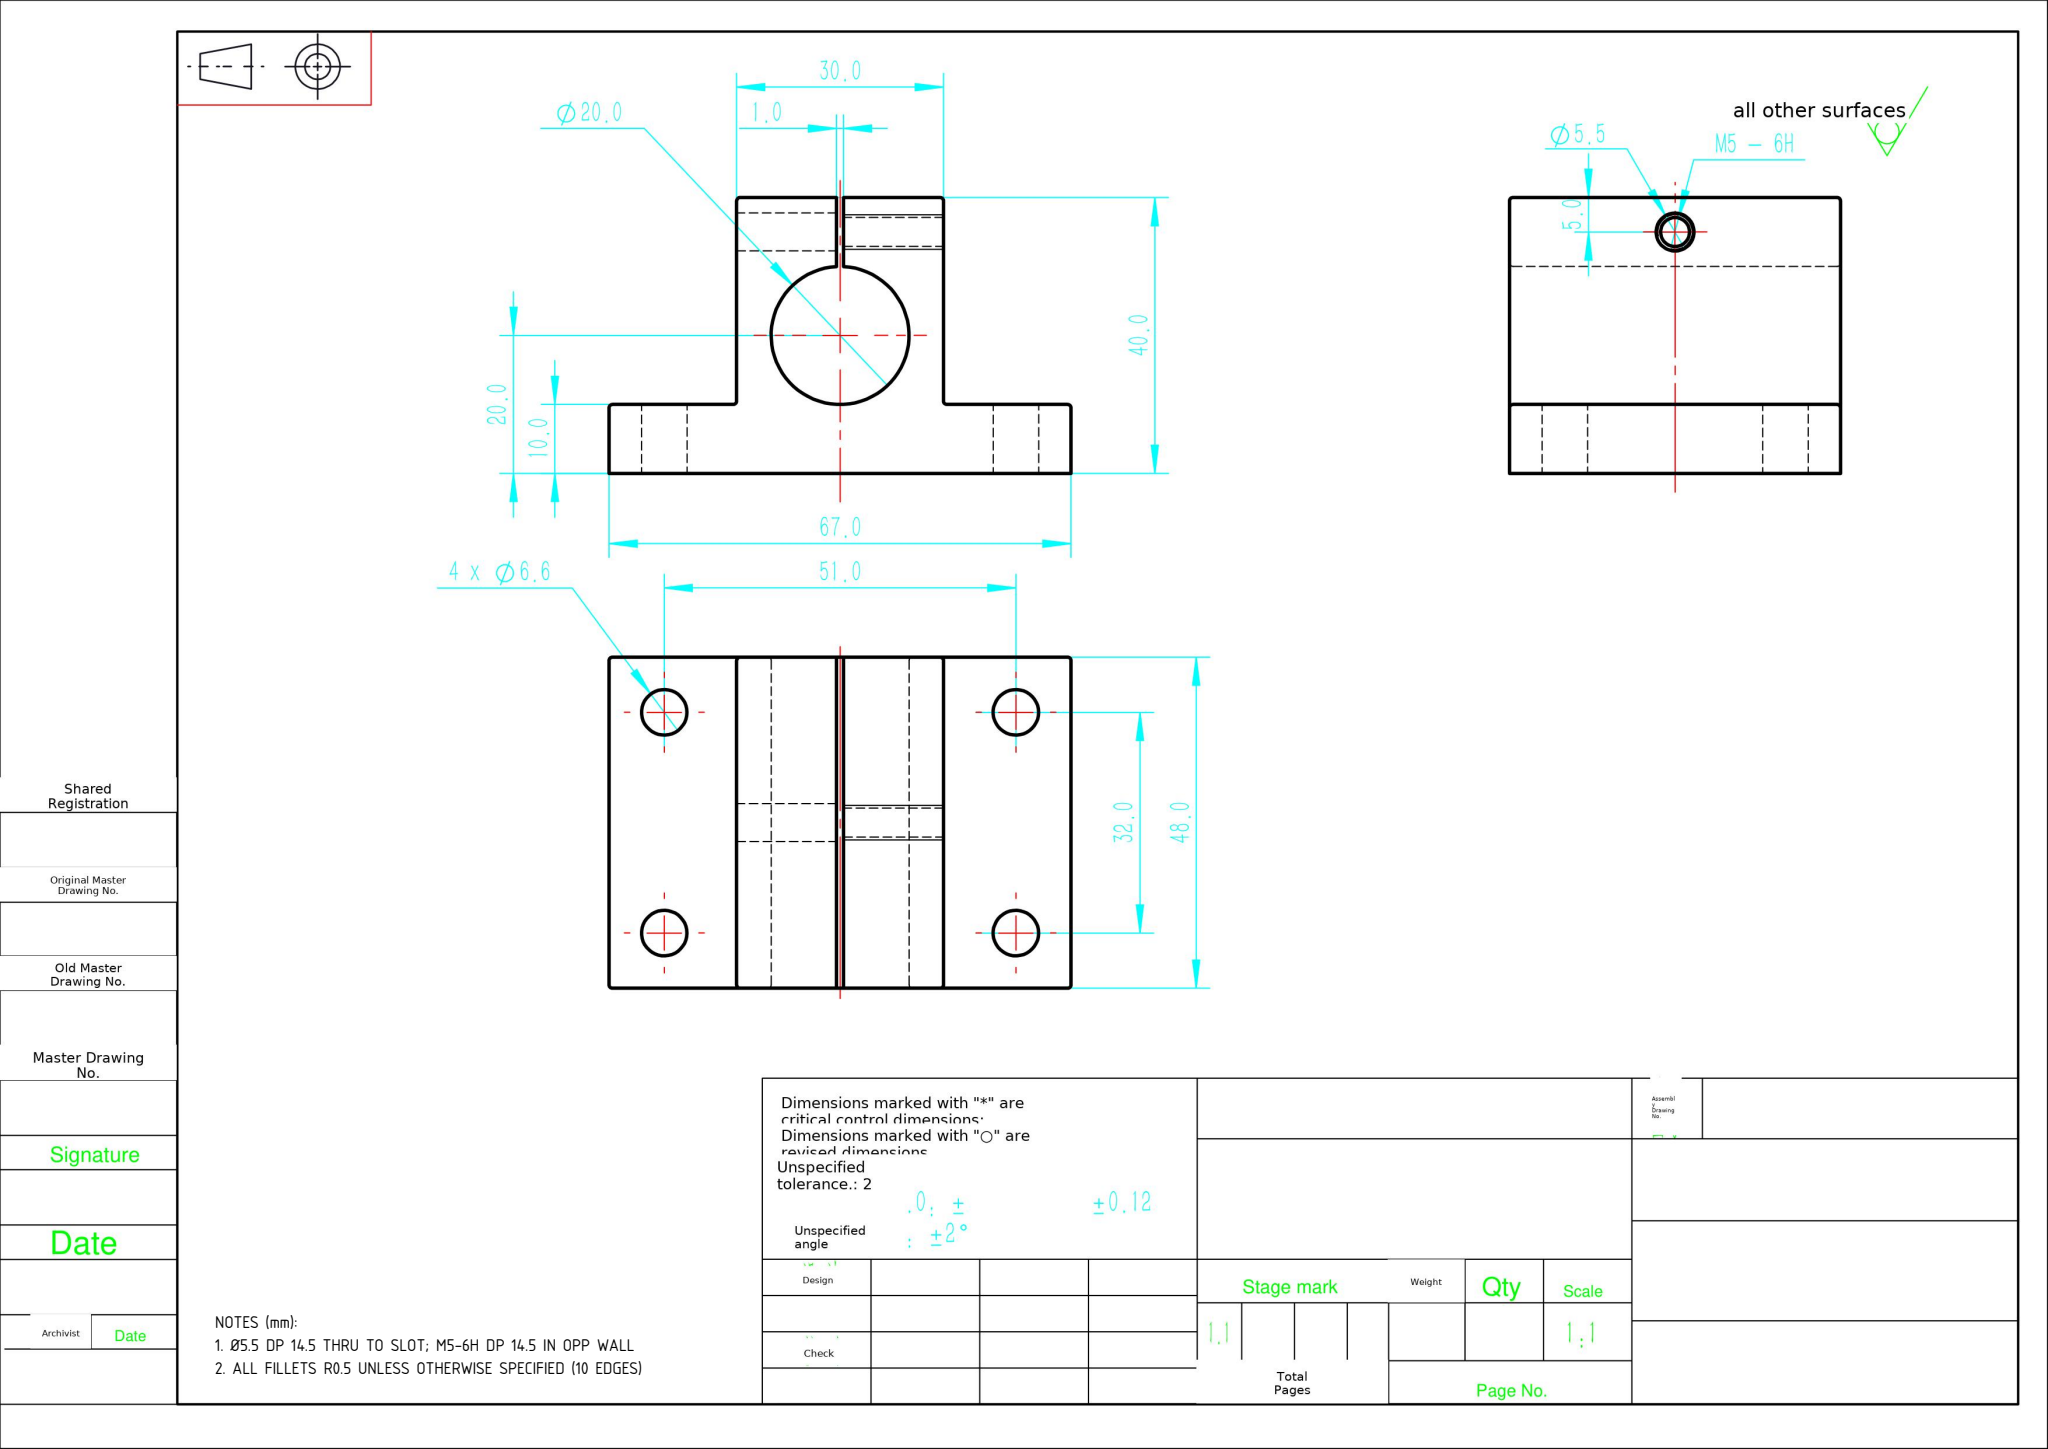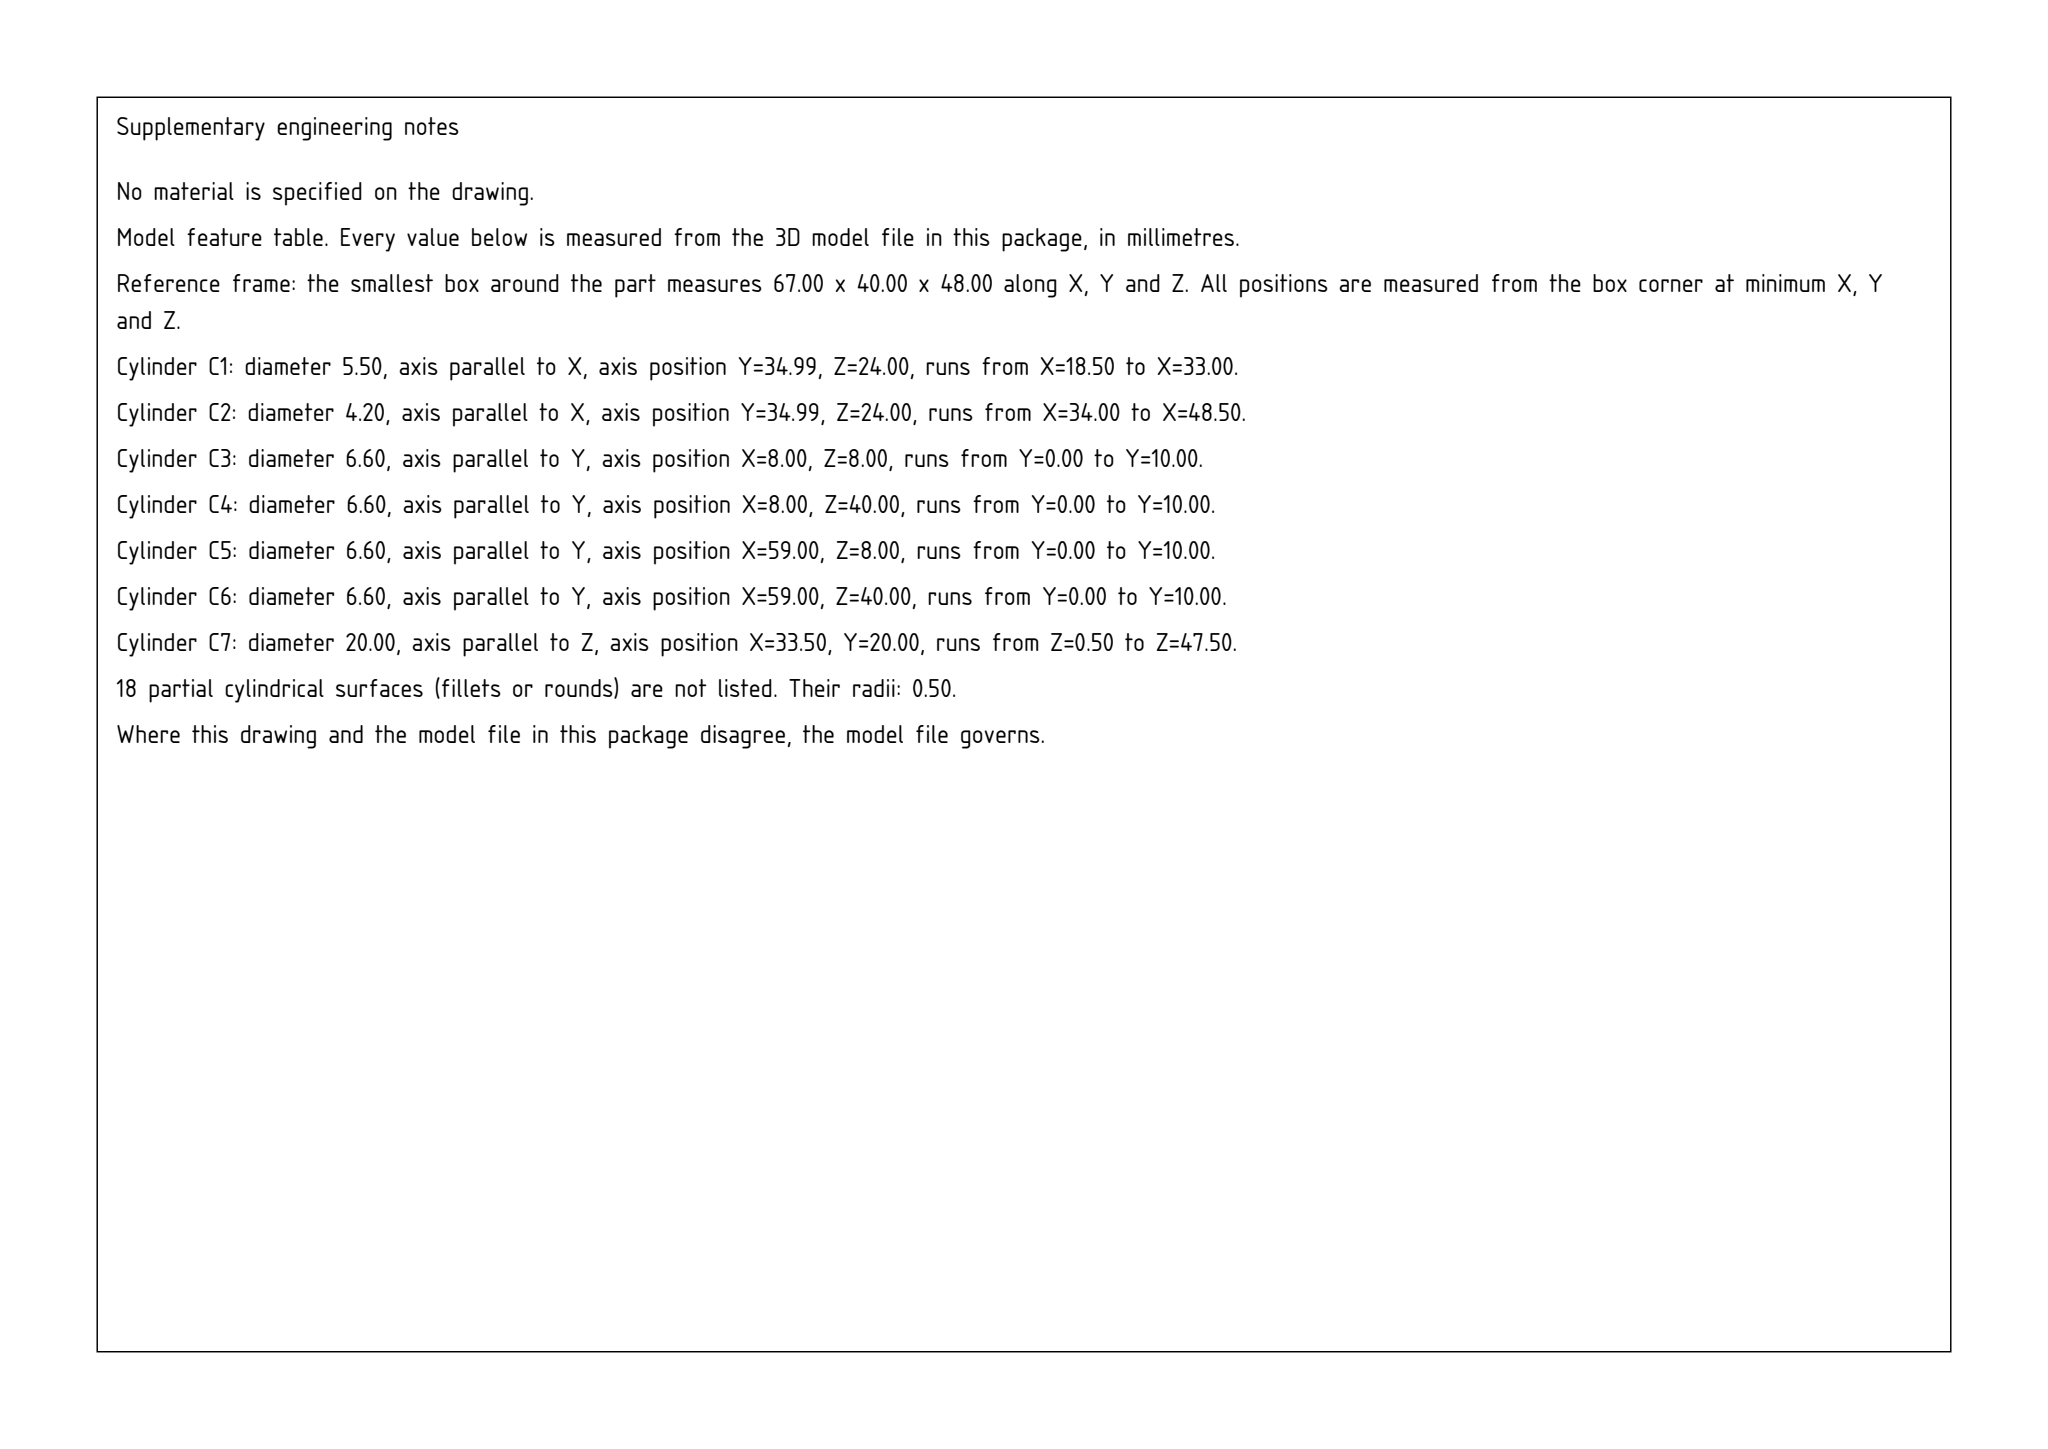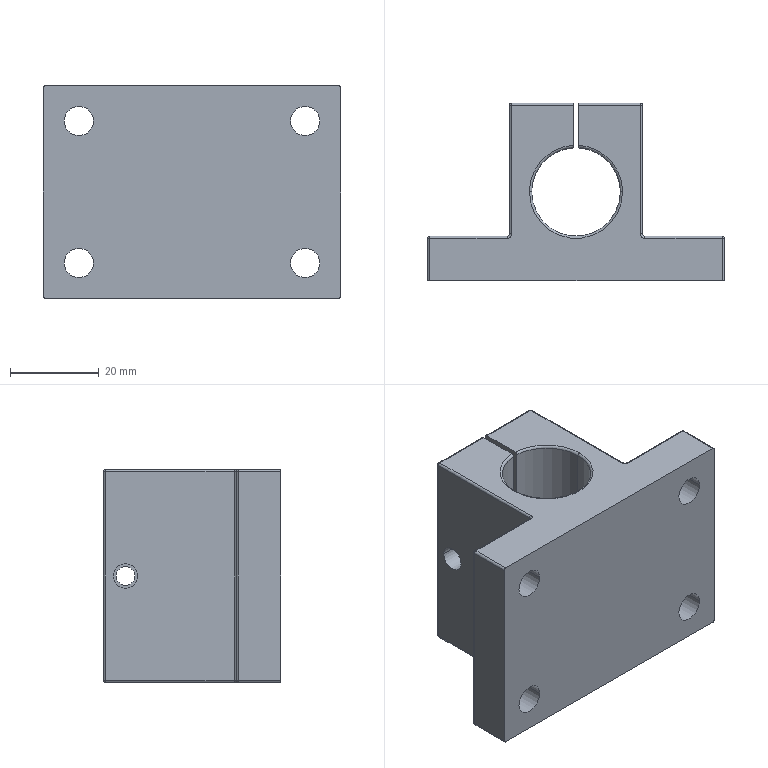Part | SolidWorks | mm | 1 solid | 68 faces | box 67 x 40 x 48 mm | volume 57859 mm3 | cylinder 37 | plane 13 | torus 10 | sphere 8 | commonest cylinder face diameters 1 x22 6.6 x8 20 x3 5.5 x2 4.2 x2
Drawing notes:
Ø5.5 DP 14.5 THRU TO SLOT; M5-6H DP 14.5 IN OPP WALL | from the solid: Ø5.5 x-cyl at y=34.99,z=24.0,len 14.5 (x18.5-33.0); Ø4.2 tap drill same axis len 14.5 (x34.0-48.5); slot faces x=33.0/34.0
ALL FILLETS R0.5 UNLESS OTHERWISE SPECIFIED (10 EDGES) | from the solid: fillet_radii: [[0.5, 10]]
build123d program:
from build123d import *

# Parameters (mm, degrees)
EXTRUDE1_DEPTH     = 24
SKETCH2_R          = 3.3
CUT_EXTRUDE1_DEPTH = 58.43
M5_TAPPED_HOLE1_D  = 4.2
FILLET1_R          = 0.5
CUT_EXTRUDE2_REACH = 59.691
SKETCH6_R          = 2.75


with BuildPart() as part:
    # Sketch1 → Extrude1 (new, symmetric)
    with BuildSketch(Plane.XY):
        with BuildLine():
            Line((33.5, -20), (-33.5, -20))
            Line((-33.5, -20), (-33.5, -10))
            Line((-33.5, -10), (-15, -10))
            Line((-15, -10), (-15, 20))
            Line((-15, 20), (-0.5, 20))
            Line((-0.5, 20), (-0.5, 9.987))
            ThreePointArc((-0.5, 9.987), (0, -10), (0.5, 9.987))
            Line((0.5, 9.987), (0.5, 20))
            Line((0.5, 20), (15, 20))
            Line((15, 20), (15, -10))
            Line((15, -10), (33.5, -10))
            Line((33.5, -10), (33.5, -20))
        make_face()
    extrude(amount=EXTRUDE1_DEPTH, both=True)

    # Sketch2 → Cut-Extrude1 (cut, through all)
    with BuildSketch(Plane.XZ.offset(20)):
        with Locations((-25.5, -16)):
            Circle(SKETCH2_R)
        with Locations((25.5, -16)):
            Circle(SKETCH2_R)
        with Locations((-25.5, 16)):
            Circle(SKETCH2_R)
        with Locations((25.5, 16)):
            Circle(SKETCH2_R)
    extrude(amount=-CUT_EXTRUDE1_DEPTH, mode=Mode.SUBTRACT)

    # M5 Tapped Hole1 (through all)
    with Locations(Plane.ZY.offset(15)):
        with Locations((0, 14.994)):
            Hole(M5_TAPPED_HOLE1_D / 2)

    # Fillet1
    fillet1_edges = [part.edges().sort_by_distance(p)[0] for p in [
        (33.5, -15, 24),
        (-24.25, -10, -24),
        (-15, 5, -24),
        (-7.75, 20, -24),
        (0, -10, -24),
        (24.25, -10, 24),
        (7.75, 20, -24),
        (15, 5, -24),
        (24.25, -10, -24),
        (33.5, -15, -24),
        (-33.5, -15, -24),
        (15, 5, 24),
        (7.75, 20, 24),
        (-33.5, -10, 0),
        (-15, -10, 0),
        (-15, 20, 0),
        (15, 20, 0),
        (15, -10, 0),
        (33.5, -10, 0),
        (0, -10, 24),
        (-7.75, 20, 24),
        (-15, 5, 24),
        (-24.25, -10, 24),
        (-33.5, -15, 24),
    ]]
    fillet(fillet1_edges, radius=FILLET1_R)

    # Sketch6 → Cut-Extrude2 (cut, up to next)
    with BuildSketch(Plane(origin=(-15, 0, 0), x_dir=(0, 0, -1), z_dir=(1, 0, 0)), mode=Mode.PRIVATE) as cut_extrude2_sk1:
        with Locations(Location((0, 14.994, 0), (0, 0, 270))):
            Circle(SKETCH6_R)
    cut_extrude2_tool1 = extrude(cut_extrude2_sk1.sketch, amount=CUT_EXTRUDE2_REACH, mode=Mode.PRIVATE) & part.part
    add(cut_extrude2_tool1.solids().sort_by_distance((-15, 14.994, 0))[0], mode=Mode.SUBTRACT)


solid = part.part